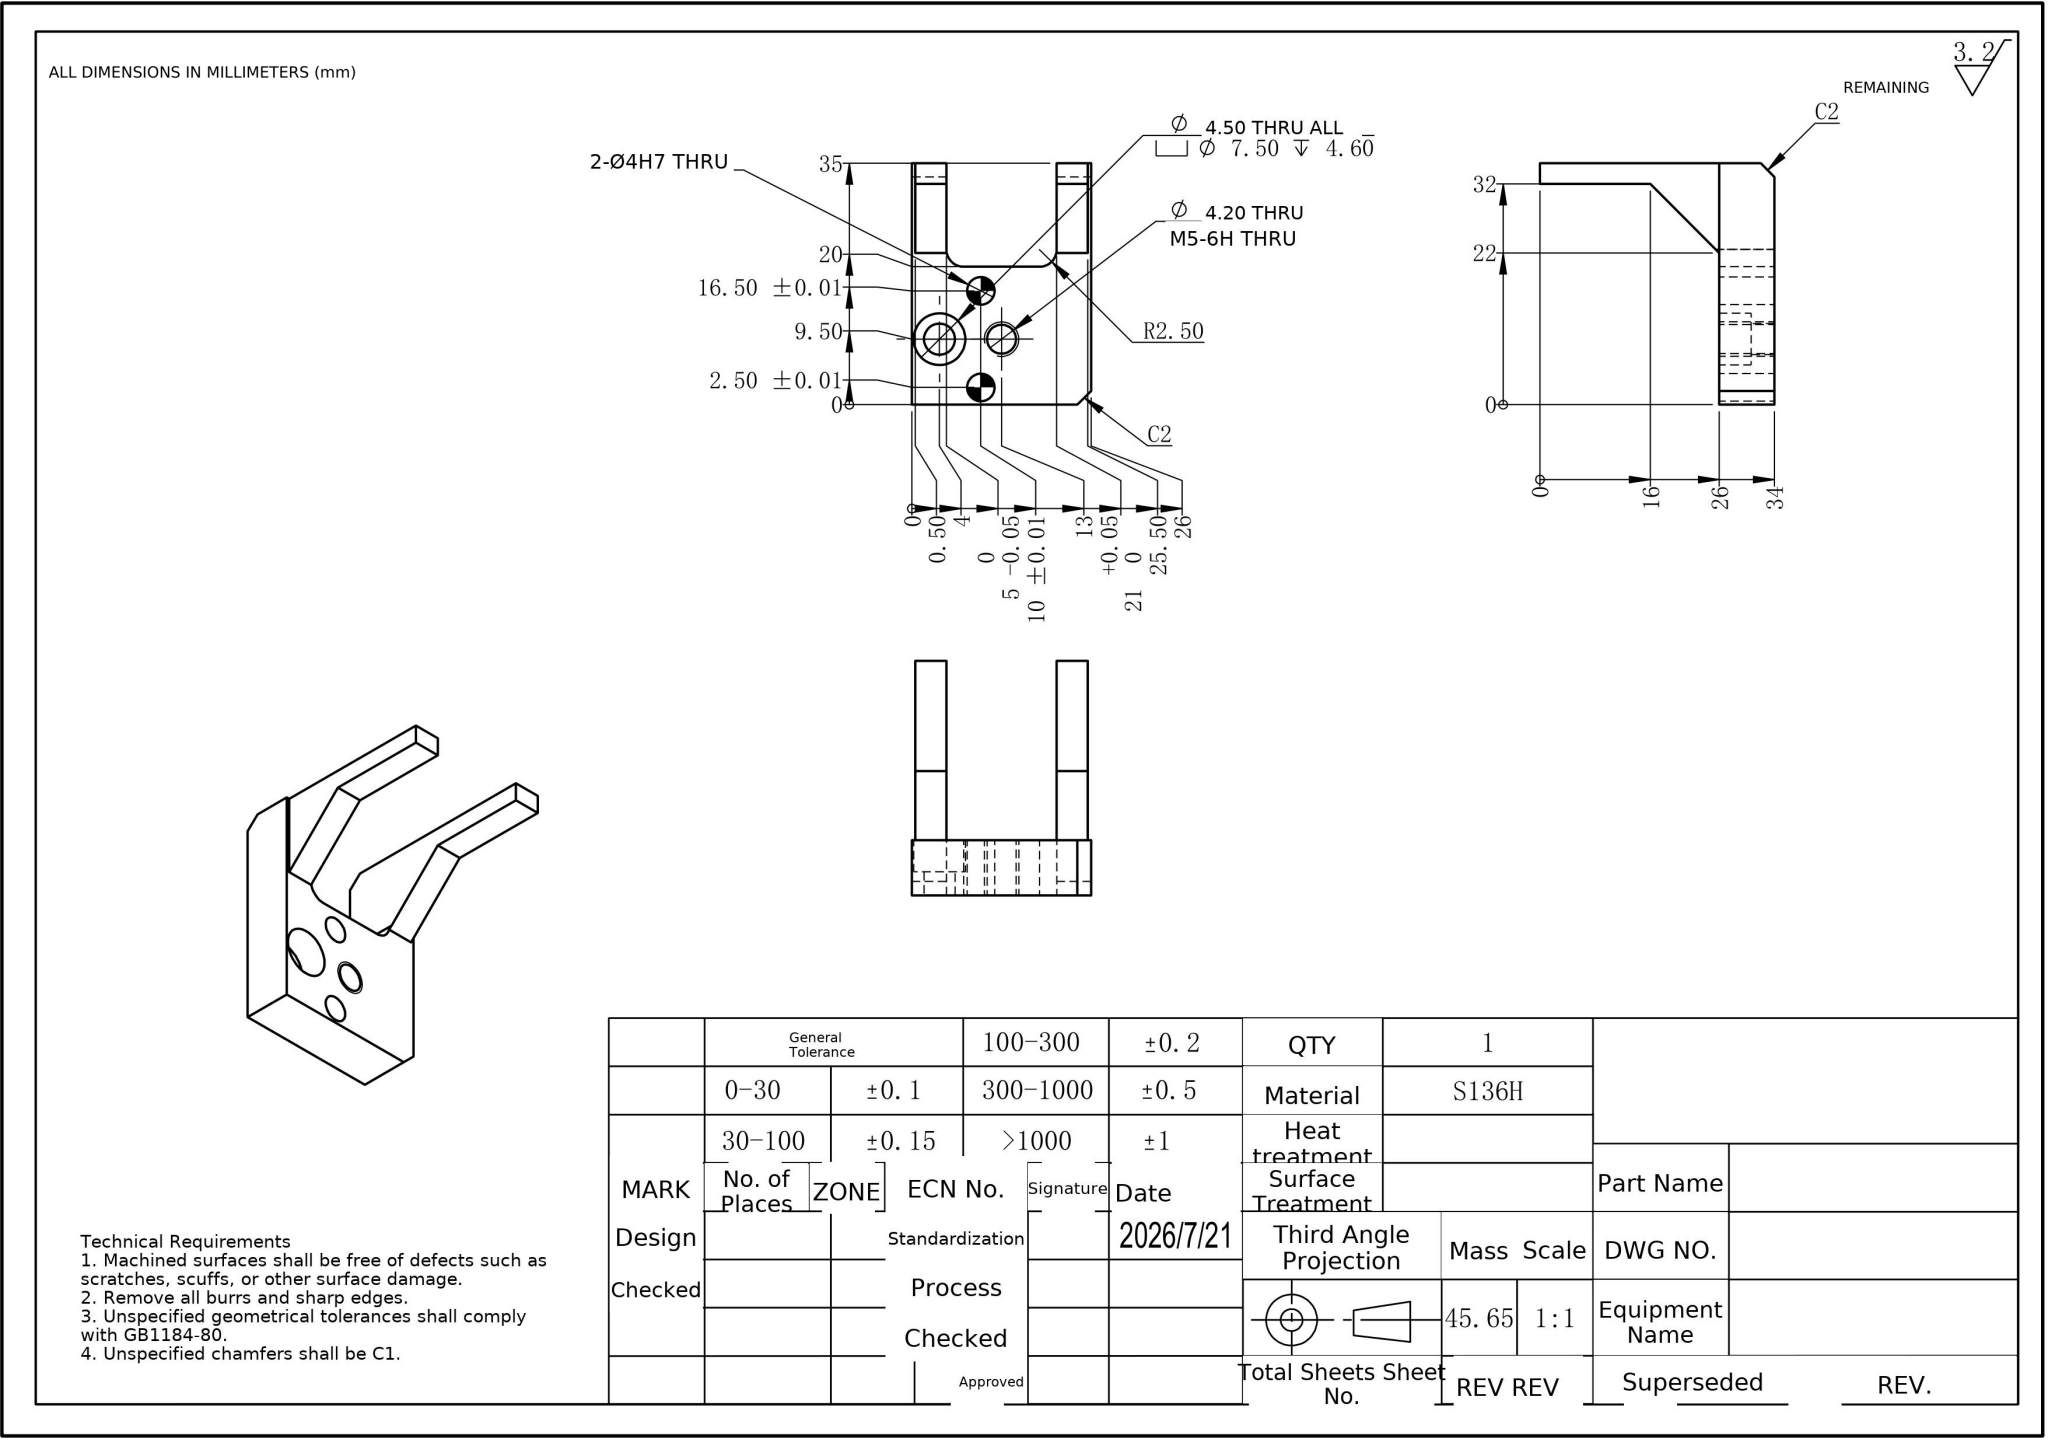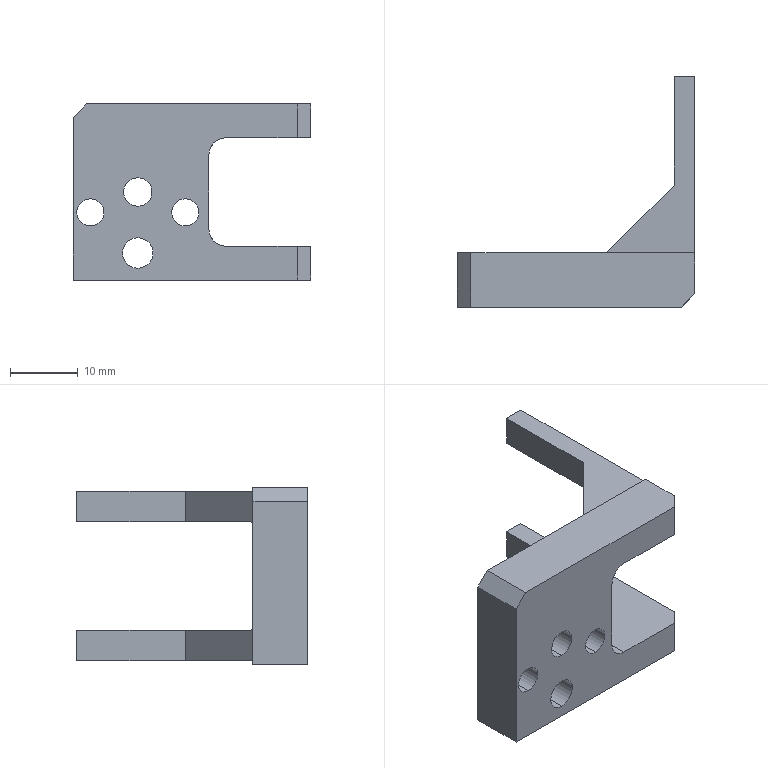Part | NX | mm | 1 solid | 34 faces | box 35 x 34 x 26 mm | volume 5928 mm3 | plane 22 | cylinder 12 | commonest cylinder face diameters 4 x4 7.5 x2 4.5 x2 4.2 x2 5 x2